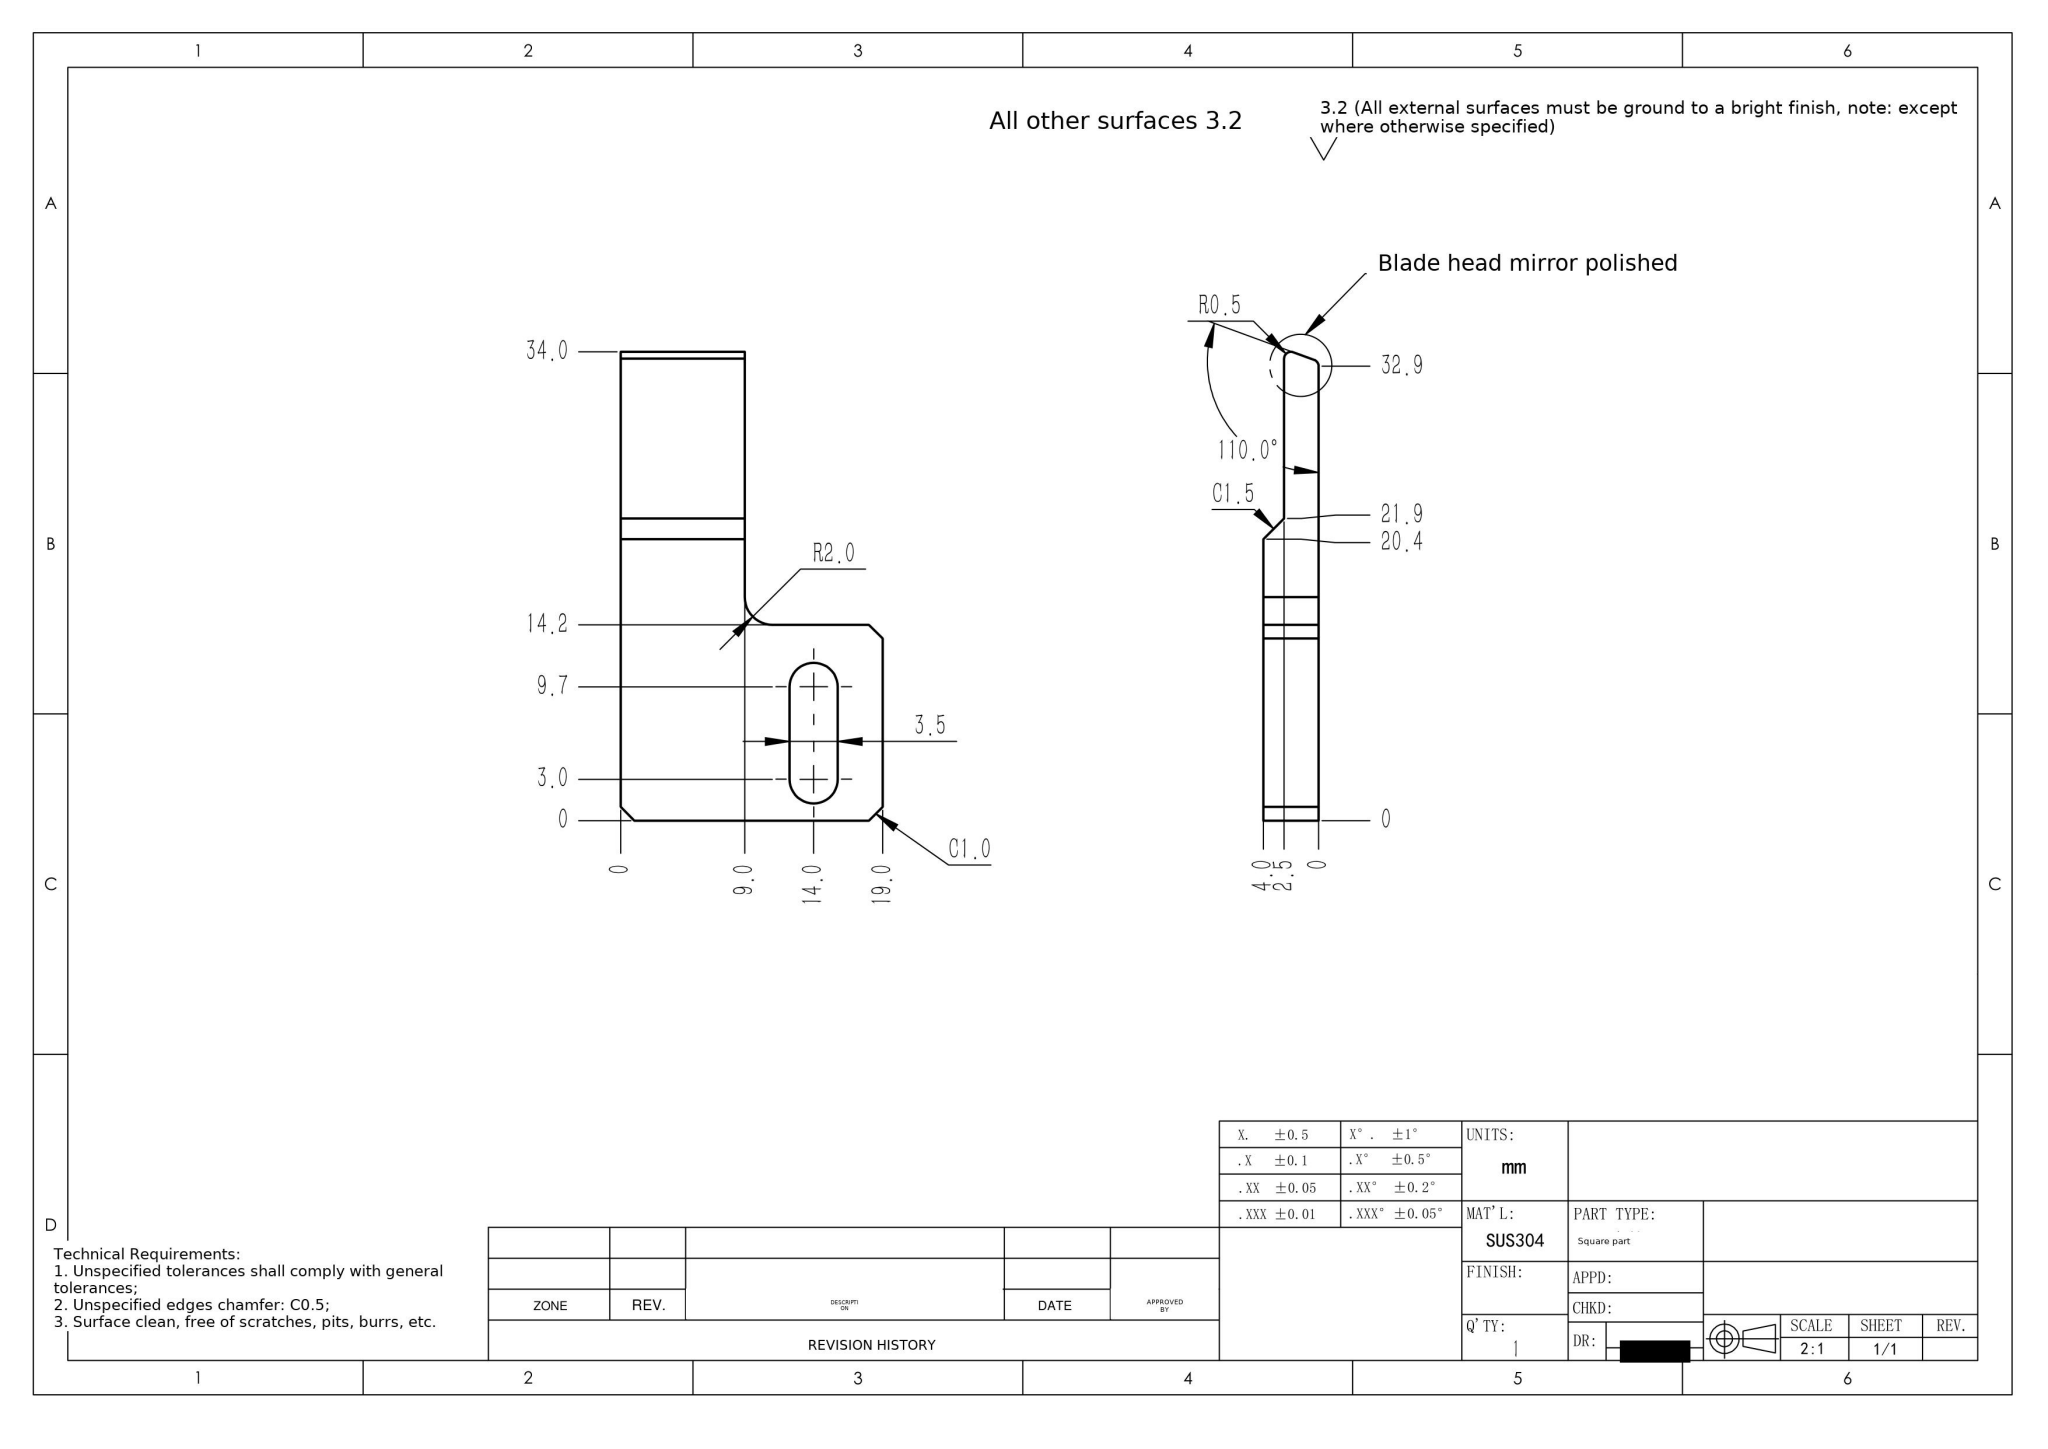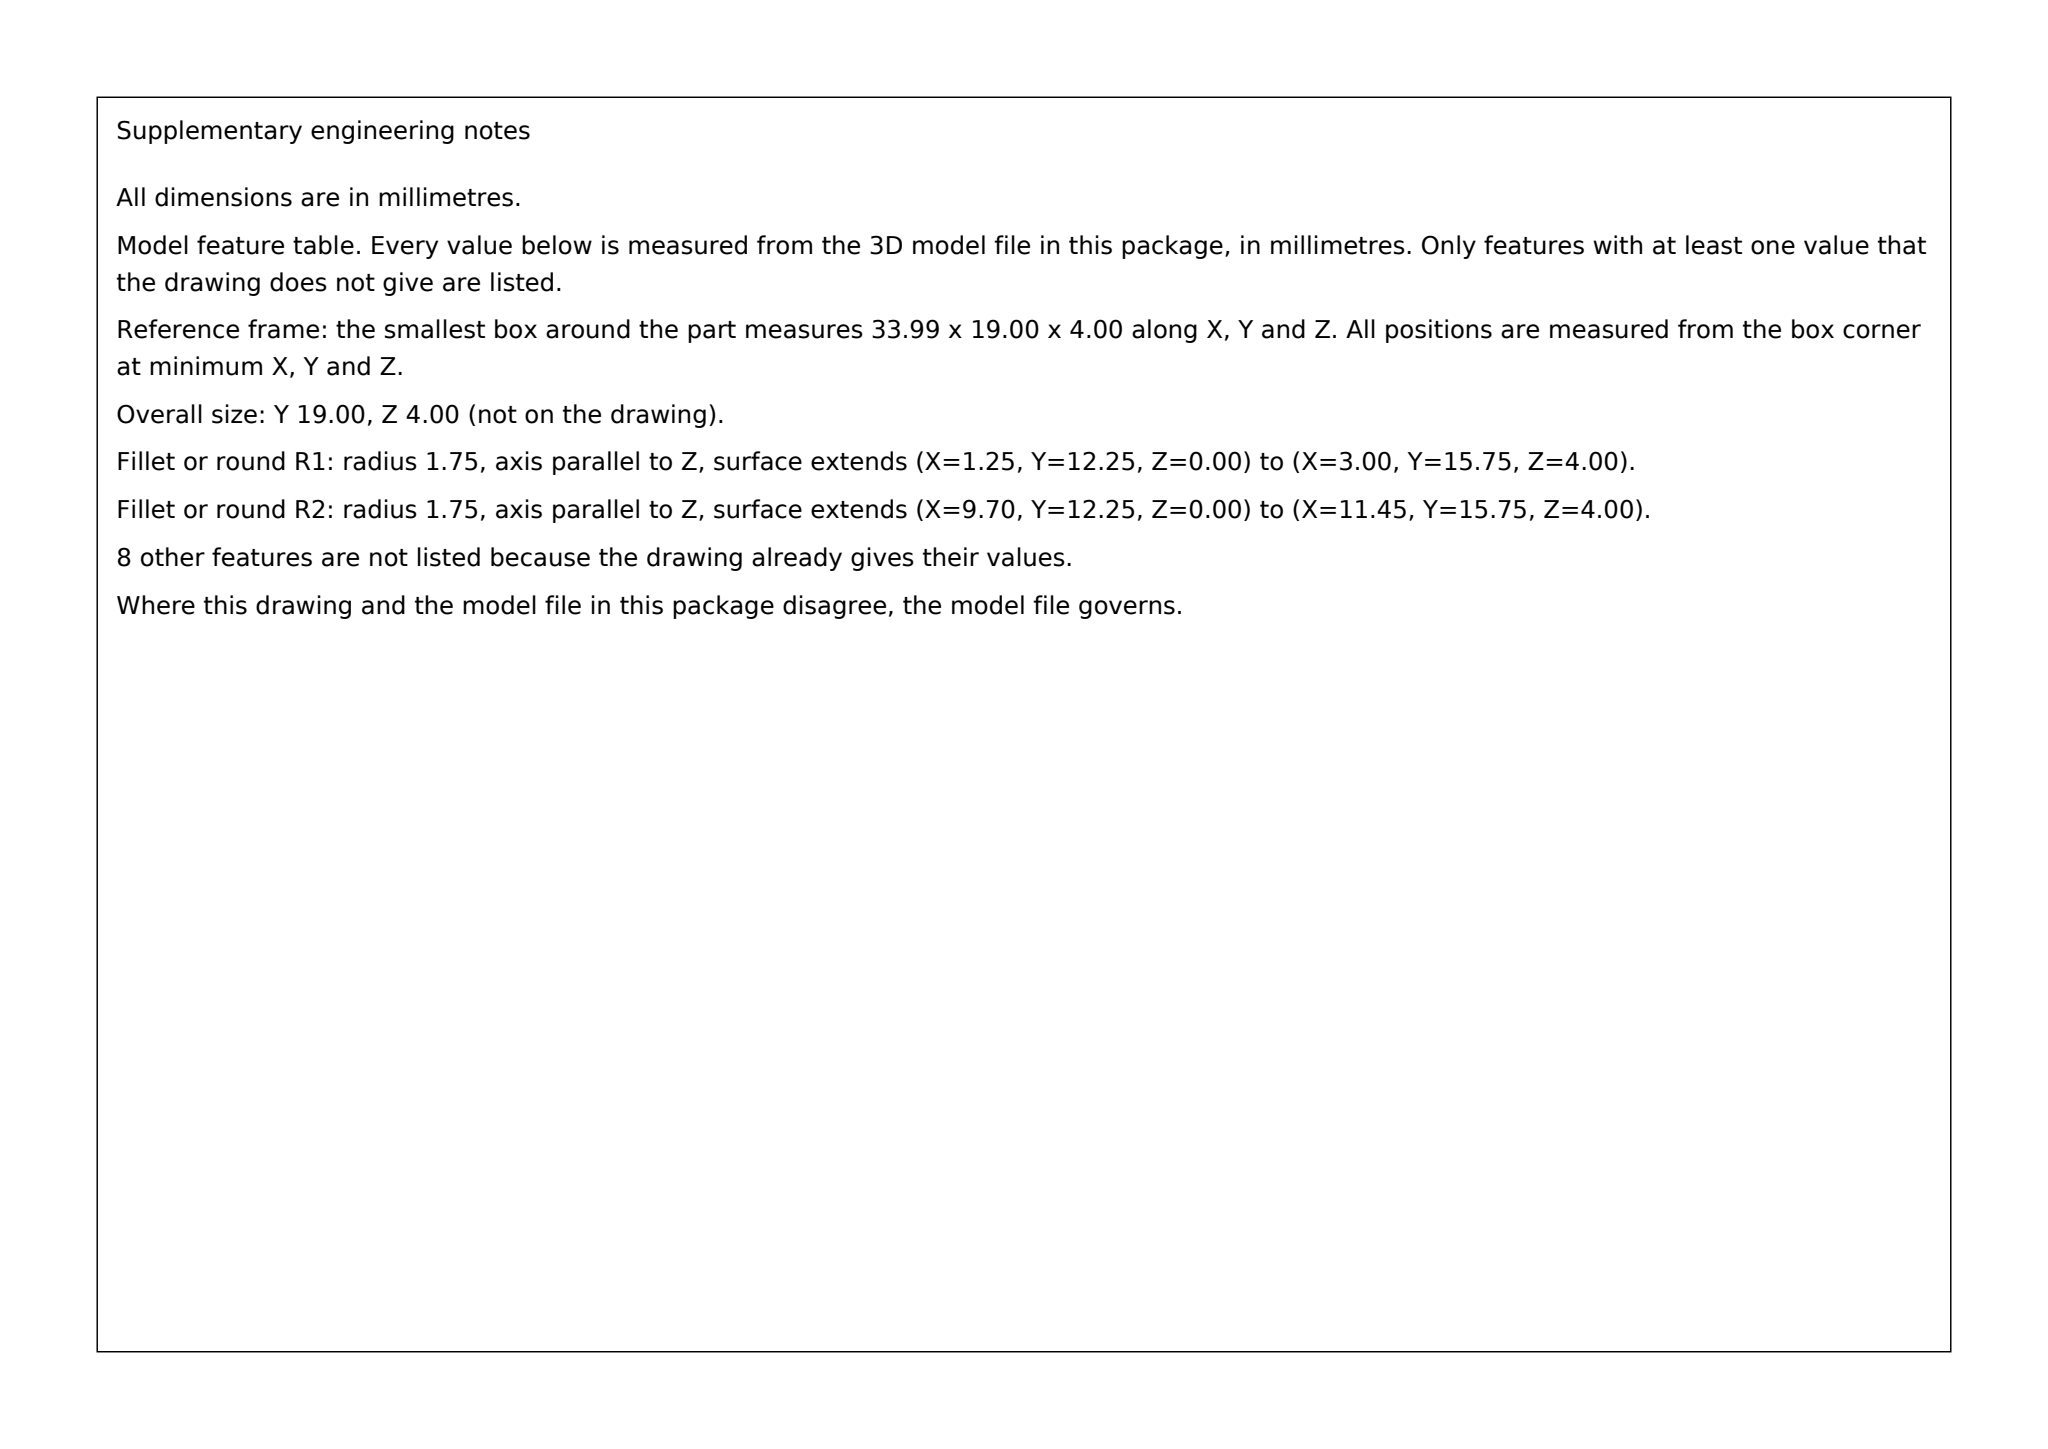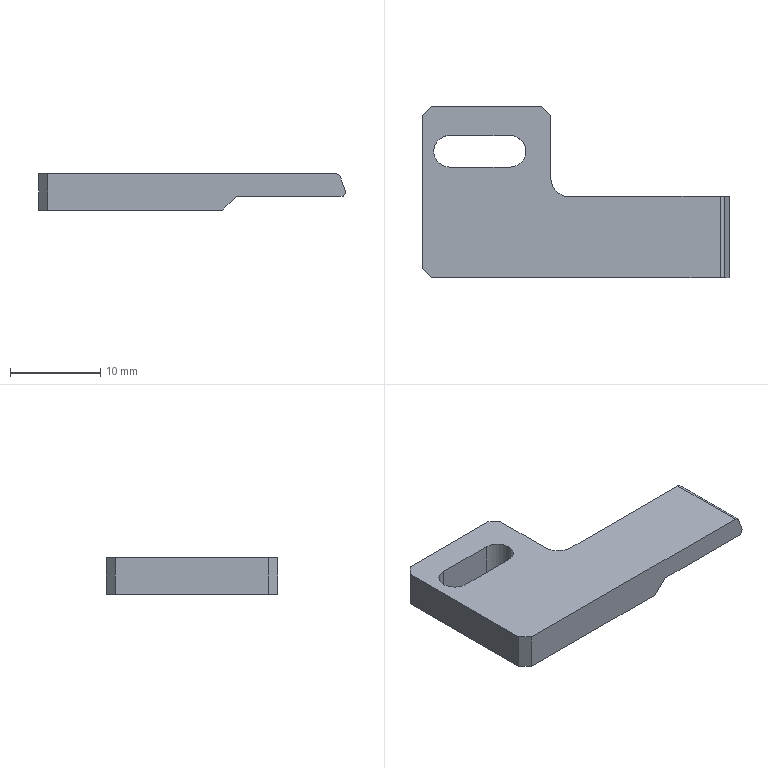Part | SolidWorks | mm | material SUS304 | 1 solid | 21 faces | box 33.99 x 19 x 4 mm | volume 1477 mm3 | plane 15 | cylinder 6 | commonest cylinder face diameters 3.5 x3 1 x2 4 x1
STEP:
#1=CARTESIAN_POINT('',(11.45,-5.,0.));
#2=VERTEX_POINT('',#1);
#3=CARTESIAN_POINT('',(9.7,-3.25,0.));
#4=VERTEX_POINT('',#3);
#5=CARTESIAN_POINT('',(9.7,-5.,0.));
#6=DIRECTION('',(0.,0.,1.));
#7=DIRECTION('',(1.,0.,0.));
#8=AXIS2_PLACEMENT_3D('',#5,#6,#7);
#9=CIRCLE('',#8,1.75);
#10=EDGE_CURVE('',#2,#4,#9,.T.);
#11=ORIENTED_EDGE('',*,*,#10,.F.);
#12=CARTESIAN_POINT('',(11.45,-5.,4.));
#13=VERTEX_POINT('',#12);
#14=CARTESIAN_POINT('',(11.45,-5.,0.));
#15=DIRECTION('',(0.,0.,1.));
#16=VECTOR('',#15,1000.);
#17=LINE('',#14,#16);
#18=EDGE_CURVE('',#2,#13,#17,.T.);
#19=ORIENTED_EDGE('',*,*,#18,.T.);
#20=CARTESIAN_POINT('',(9.7,-3.25,4.));
#21=VERTEX_POINT('',#20);
#22=CARTESIAN_POINT('',(9.7,-5.,4.));
#23=DIRECTION('',(0.,0.,1.));
#24=DIRECTION('',(1.,0.,0.));
#25=AXIS2_PLACEMENT_3D('',#22,#23,#24);
#26=CIRCLE('',#25,1.75);
#27=EDGE_CURVE('',#13,#21,#26,.T.);
#28=ORIENTED_EDGE('',*,*,#27,.T.);
#29=CARTESIAN_POINT('',(9.7,-3.25,0.));
#30=DIRECTION('',(0.,0.,1.));
#31=VECTOR('',#30,1000.);
#32=LINE('',#29,#31);
#33=EDGE_CURVE('',#4,#21,#32,.T.);
#34=ORIENTED_EDGE('',*,*,#33,.F.);
#35=EDGE_LOOP('',(#11,#19,#28,#34));
#36=FACE_OUTER_BOUND('',#35,.T.);
#37=CARTESIAN_POINT('',(9.7,-5.,0.));
#38=DIRECTION('',(0.,0.,1.));
#39=DIRECTION('',(1.,0.,0.));
#40=AXIS2_PLACEMENT_3D('',#37,#38,#39);
#41=CYLINDRICAL_SURFACE('',#40,1.75);
#42=ADVANCED_FACE('',(#36),#41,.F.);
#43=CARTESIAN_POINT('',(0.,-1.,4.));
#44=VERTEX_POINT('',#43);
#45=CARTESIAN_POINT('',(0.,-18.,4.));
#46=VERTEX_POINT('',#45);
#47=CARTESIAN_POINT('',(0.,0.,4.));
#48=DIRECTION('',(0.,-1.,0.));
#49=VECTOR('',#48,1000.);
#50=LINE('',#47,#49);
#51=EDGE_CURVE('',#44,#46,#50,.T.);
#52=ORIENTED_EDGE('',*,*,#51,.F.);
#53=CARTESIAN_POINT('',(0.,-1.,0.));
#54=VERTEX_POINT('',#53);
#55=CARTESIAN_POINT('',(0.,-1.,4.));
#56=DIRECTION('',(0.,0.,-1.));
#57=VECTOR('',#56,1000.);
#58=LINE('',#55,#57);
#59=EDGE_CURVE('',#44,#54,#58,.T.);
#60=ORIENTED_EDGE('',*,*,#59,.T.);
#61=CARTESIAN_POINT('',(0.,-18.,0.));
#62=VERTEX_POINT('',#61);
#63=CARTESIAN_POINT('',(0.,0.,0.));
#64=DIRECTION('',(0.,-1.,0.));
#65=VECTOR('',#64,1000.);
#66=LINE('',#63,#65);
#67=EDGE_CURVE('',#54,#62,#66,.T.);
#68=ORIENTED_EDGE('',*,*,#67,.T.);
#69=CARTESIAN_POINT('',(0.,-18.,4.));
#70=DIRECTION('',(0.,0.,1.));
#71=VECTOR('',#70,1000.);
#72=LINE('',#69,#71);
#73=EDGE_CURVE('',#62,#46,#72,.T.);
#74=ORIENTED_EDGE('',*,*,#73,.T.);
#75=EDGE_LOOP('',(#52,#60,#68,#74));
#76=FACE_OUTER_BOUND('',#75,.T.);
#77=CARTESIAN_POINT('',(0.,0.,4.));
#78=DIRECTION('',(1.,0.,0.));
#79=DIRECTION('',(0.,0.,-1.));
#80=AXIS2_PLACEMENT_3D('',#77,#78,#79);
#81=PLANE('',#80);
#82=ADVANCED_FACE('',(#76),#81,.F.);
#83=CARTESIAN_POINT('',(1.,-19.,4.));
#84=VERTEX_POINT('',#83);
#85=CARTESIAN_POINT('',(32.94,-19.,4.));
#86=VERTEX_POINT('',#85);
#87=CARTESIAN_POINT('',(0.,-19.,4.));
#88=DIRECTION('',(1.,0.,0.));
#89=VECTOR('',#88,1000.);
#90=LINE('',#87,#89);
#91=EDGE_CURVE('',#84,#86,#90,.T.);
#92=ORIENTED_EDGE('',*,*,#91,.F.);
#93=CARTESIAN_POINT('',(1.,-19.,0.));
#94=VERTEX_POINT('',#93);
#95=CARTESIAN_POINT('',(1.,-19.,4.));
#96=DIRECTION('',(0.,0.,-1.));
#97=VECTOR('',#96,1000.);
#98=LINE('',#95,#97);
#99=EDGE_CURVE('',#84,#94,#98,.T.);
#100=ORIENTED_EDGE('',*,*,#99,.T.);
#101=CARTESIAN_POINT('',(20.4,-19.,0.));
#102=VERTEX_POINT('',#101);
#103=CARTESIAN_POINT('',(0.,-19.,0.));
#104=DIRECTION('',(1.,0.,0.));
#105=VECTOR('',#104,1000.);
#106=LINE('',#103,#105);
#107=EDGE_CURVE('',#94,#102,#106,.T.);
#108=ORIENTED_EDGE('',*,*,#107,.T.);
#109=CARTESIAN_POINT('',(21.9,-19.,1.5));
#110=VERTEX_POINT('',#109);
#111=CARTESIAN_POINT('',(12.2,-19.,-8.2));
#112=DIRECTION('',(0.7071,0.,0.7071));
#113=VECTOR('',#112,1000.);
#114=LINE('',#111,#113);
#115=EDGE_CURVE('',#102,#110,#114,.T.);
#116=ORIENTED_EDGE('',*,*,#115,.T.);
#117=CARTESIAN_POINT('',(33.486,-19.,1.5));
#118=VERTEX_POINT('',#117);
#119=CARTESIAN_POINT('',(34.2,-19.,1.5));
#120=DIRECTION('',(-1.,0.,-0.));
#121=VECTOR('',#120,1000.);
#122=LINE('',#119,#121);
#123=EDGE_CURVE('',#118,#110,#122,.T.);
#124=ORIENTED_EDGE('',*,*,#123,.F.);
#125=CARTESIAN_POINT('',(33.956,-19.,2.171));
#126=VERTEX_POINT('',#125);
#127=CARTESIAN_POINT('',(33.486,-19.,2.));
#128=DIRECTION('',(0.,-1.,0.));
#129=DIRECTION('',(-0.,0.,1.));
#130=AXIS2_PLACEMENT_3D('',#127,#128,#129);
#131=CIRCLE('',#130,0.5);
#132=EDGE_CURVE('',#118,#126,#131,.T.);
#133=ORIENTED_EDGE('',*,*,#132,.T.);
#134=CARTESIAN_POINT('',(33.41,-19.,3.671));
#135=VERTEX_POINT('',#134);
#136=CARTESIAN_POINT('',(34.2,-19.,1.5));
#137=DIRECTION('',(0.342,0.,-0.9397));
#138=VECTOR('',#137,1000.);
#139=LINE('',#136,#138);
#140=EDGE_CURVE('',#135,#126,#139,.T.);
#141=ORIENTED_EDGE('',*,*,#140,.F.);
#142=CARTESIAN_POINT('',(32.94,-19.,3.5));
#143=DIRECTION('',(0.,-1.,0.));
#144=DIRECTION('',(0.,0.,1.));
#145=AXIS2_PLACEMENT_3D('',#142,#143,#144);
#146=CIRCLE('',#145,0.5);
#147=EDGE_CURVE('',#135,#86,#146,.T.);
#148=ORIENTED_EDGE('',*,*,#147,.T.);
#149=EDGE_LOOP('',(#92,#100,#108,#116,#124,#133,#141,#148));
#150=FACE_OUTER_BOUND('',#149,.T.);
#151=CARTESIAN_POINT('',(0.,-19.,4.));
#152=DIRECTION('',(0.,1.,0.));
#153=DIRECTION('',(0.,0.,1.));
#154=AXIS2_PLACEMENT_3D('',#151,#152,#153);
#155=PLANE('',#154);
#156=ADVANCED_FACE('',(#150),#155,.F.);
#157=CARTESIAN_POINT('',(13.2,0.,4.));
#158=VERTEX_POINT('',#157);
#159=CARTESIAN_POINT('',(1.,0.,4.));
#160=VERTEX_POINT('',#159);
#161=CARTESIAN_POINT('',(0.,0.,4.));
#162=DIRECTION('',(-1.,0.,0.));
#163=VECTOR('',#162,1000.);
#164=LINE('',#161,#163);
#165=EDGE_CURVE('',#158,#160,#164,.T.);
#166=ORIENTED_EDGE('',*,*,#165,.F.);
#167=CARTESIAN_POINT('',(13.2,0.,0.));
#168=VERTEX_POINT('',#167);
#169=CARTESIAN_POINT('',(13.2,0.,4.));
#170=DIRECTION('',(0.,0.,-1.));
#171=VECTOR('',#170,1000.);
#172=LINE('',#169,#171);
#173=EDGE_CURVE('',#158,#168,#172,.T.);
#174=ORIENTED_EDGE('',*,*,#173,.T.);
#175=CARTESIAN_POINT('',(1.,0.,0.));
#176=VERTEX_POINT('',#175);
#177=CARTESIAN_POINT('',(0.,0.,0.));
#178=DIRECTION('',(-1.,0.,0.));
#179=VECTOR('',#178,1000.);
#180=LINE('',#177,#179);
#181=EDGE_CURVE('',#168,#176,#180,.T.);
#182=ORIENTED_EDGE('',*,*,#181,.T.);
#183=CARTESIAN_POINT('',(1.,0.,4.));
#184=DIRECTION('',(0.,0.,1.));
#185=VECTOR('',#184,1000.);
#186=LINE('',#183,#185);
#187=EDGE_CURVE('',#176,#160,#186,.T.);
#188=ORIENTED_EDGE('',*,*,#187,.T.);
#189=EDGE_LOOP('',(#166,#174,#182,#188));
#190=FACE_OUTER_BOUND('',#189,.T.);
#191=CARTESIAN_POINT('',(0.,0.,4.));
#192=DIRECTION('',(0.,-1.,0.));
#193=DIRECTION('',(0.,0.,-1.));
#194=AXIS2_PLACEMENT_3D('',#191,#192,#193);
#195=PLANE('',#194);
#196=ADVANCED_FACE('',(#190),#195,.F.);
#197=CARTESIAN_POINT('',(14.2,-1.,4.));
#198=VERTEX_POINT('',#197);
#199=CARTESIAN_POINT('',(14.2,-8.,4.));
#200=VERTEX_POINT('',#199);
#201=CARTESIAN_POINT('',(14.2,-0.,4.));
#202=DIRECTION('',(0.,-1.,0.));
#203=VECTOR('',#202,1000.);
#204=LINE('',#201,#203);
#205=EDGE_CURVE('',#198,#200,#204,.T.);
#206=ORIENTED_EDGE('',*,*,#205,.F.);
#207=CARTESIAN_POINT('',(6.6,6.6,4.));
#208=DIRECTION('',(-0.7071,0.7071,0.));
#209=VECTOR('',#208,1000.);
#210=LINE('',#207,#209);
#211=EDGE_CURVE('',#198,#158,#210,.T.);
#212=ORIENTED_EDGE('',*,*,#211,.T.);
#213=ORIENTED_EDGE('',*,*,#165,.T.);
#214=CARTESIAN_POINT('',(0.5,-0.5,4.));
#215=DIRECTION('',(-0.7071,-0.7071,0.));
#216=VECTOR('',#215,1000.);
#217=LINE('',#214,#216);
#218=EDGE_CURVE('',#160,#44,#217,.T.);
#219=ORIENTED_EDGE('',*,*,#218,.T.);
#220=ORIENTED_EDGE('',*,*,#51,.T.);
#221=CARTESIAN_POINT('',(-9.,-9.,4.));
#222=DIRECTION('',(0.7071,-0.7071,0.));
#223=VECTOR('',#222,1000.);
#224=LINE('',#221,#223);
#225=EDGE_CURVE('',#46,#84,#224,.T.);
#226=ORIENTED_EDGE('',*,*,#225,.T.);
#227=ORIENTED_EDGE('',*,*,#91,.T.);
#228=CARTESIAN_POINT('',(32.94,-10.,4.));
#229=VERTEX_POINT('',#228);
#230=CARTESIAN_POINT('',(32.94,-10.,4.));
#231=DIRECTION('',(0.,1.,0.));
#232=VECTOR('',#231,1000.);
#233=LINE('',#230,#232);
#234=EDGE_CURVE('',#86,#229,#233,.T.);
#235=ORIENTED_EDGE('',*,*,#234,.T.);
#236=CARTESIAN_POINT('',(16.2,-10.,4.));
#237=VERTEX_POINT('',#236);
#238=CARTESIAN_POINT('',(34.2,-10.,4.));
#239=DIRECTION('',(1.,0.,0.));
#240=VECTOR('',#239,1000.);
#241=LINE('',#238,#240);
#242=EDGE_CURVE('',#237,#229,#241,.T.);
#243=ORIENTED_EDGE('',*,*,#242,.F.);
#244=CARTESIAN_POINT('',(16.2,-8.,4.));
#245=DIRECTION('',(0.,0.,-1.));
#246=DIRECTION('',(1.,0.,0.));
#247=AXIS2_PLACEMENT_3D('',#244,#245,#246);
#248=CIRCLE('',#247,2.);
#249=EDGE_CURVE('',#237,#200,#248,.T.);
#250=ORIENTED_EDGE('',*,*,#249,.T.);
#251=EDGE_LOOP('',(#206,#212,#213,#219,#220,#226,#227,#235,#243,#250));
#252=FACE_OUTER_BOUND('',#251,.T.);
#253=CARTESIAN_POINT('',(3.,-3.25,4.));
#254=VERTEX_POINT('',#253);
#255=CARTESIAN_POINT('',(3.,-6.75,4.));
#256=VERTEX_POINT('',#255);
#257=CARTESIAN_POINT('',(3.,-5.,4.));
#258=DIRECTION('',(0.,0.,1.));
#259=DIRECTION('',(1.,0.,0.));
#260=AXIS2_PLACEMENT_3D('',#257,#258,#259);
#261=CIRCLE('',#260,1.75);
#262=EDGE_CURVE('',#254,#256,#261,.T.);
#263=ORIENTED_EDGE('',*,*,#262,.F.);
#264=CARTESIAN_POINT('',(3.,-3.25,4.));
#265=DIRECTION('',(-1.,0.,0.));
#266=VECTOR('',#265,1000.);
#267=LINE('',#264,#266);
#268=EDGE_CURVE('',#21,#254,#267,.T.);
#269=ORIENTED_EDGE('',*,*,#268,.F.);
#270=ORIENTED_EDGE('',*,*,#27,.F.);
#271=CARTESIAN_POINT('',(9.7,-6.75,4.));
#272=VERTEX_POINT('',#271);
#273=CARTESIAN_POINT('',(9.7,-5.,4.));
#274=DIRECTION('',(0.,0.,1.));
#275=DIRECTION('',(1.,0.,0.));
#276=AXIS2_PLACEMENT_3D('',#273,#274,#275);
#277=CIRCLE('',#276,1.75);
#278=EDGE_CURVE('',#272,#13,#277,.T.);
#279=ORIENTED_EDGE('',*,*,#278,.F.);
#280=CARTESIAN_POINT('',(3.,-6.75,4.));
#281=DIRECTION('',(1.,0.,0.));
#282=VECTOR('',#281,1000.);
#283=LINE('',#280,#282);
#284=EDGE_CURVE('',#256,#272,#283,.T.);
#285=ORIENTED_EDGE('',*,*,#284,.F.);
#286=EDGE_LOOP('',(#263,#269,#270,#279,#285));
#287=FACE_BOUND('',#286,.T.);
#288=CARTESIAN_POINT('',(0.,0.,4.));
#289=DIRECTION('',(0.,0.,1.));
#290=DIRECTION('',(1.,0.,0.));
#291=AXIS2_PLACEMENT_3D('',#288,#289,#290);
#292=PLANE('',#291);
#293=ADVANCED_FACE('',(#252,#287),#292,.T.);
#294=CARTESIAN_POINT('',(3.,-3.25,0.));
#295=VERTEX_POINT('',#294);
#296=CARTESIAN_POINT('',(3.,-3.25,0.));
#297=DIRECTION('',(-1.,0.,0.));
#298=VECTOR('',#297,1000.);
#299=LINE('',#296,#298);
#300=EDGE_CURVE('',#4,#295,#299,.T.);
#301=ORIENTED_EDGE('',*,*,#300,.T.);
#302=CARTESIAN_POINT('',(3.,-6.75,0.));
#303=VERTEX_POINT('',#302);
#304=CARTESIAN_POINT('',(3.,-5.,0.));
#305=DIRECTION('',(0.,0.,1.));
#306=DIRECTION('',(1.,0.,0.));
#307=AXIS2_PLACEMENT_3D('',#304,#305,#306);
#308=CIRCLE('',#307,1.75);
#309=EDGE_CURVE('',#295,#303,#308,.T.);
#310=ORIENTED_EDGE('',*,*,#309,.T.);
#311=CARTESIAN_POINT('',(9.7,-6.75,0.));
#312=VERTEX_POINT('',#311);
#313=CARTESIAN_POINT('',(3.,-6.75,0.));
#314=DIRECTION('',(1.,0.,0.));
#315=VECTOR('',#314,1000.);
#316=LINE('',#313,#315);
#317=EDGE_CURVE('',#303,#312,#316,.T.);
#318=ORIENTED_EDGE('',*,*,#317,.T.);
#319=CARTESIAN_POINT('',(9.7,-5.,0.));
#320=DIRECTION('',(0.,0.,1.));
#321=DIRECTION('',(1.,0.,0.));
#322=AXIS2_PLACEMENT_3D('',#319,#320,#321);
#323=CIRCLE('',#322,1.75);
#324=EDGE_CURVE('',#312,#2,#323,.T.);
#325=ORIENTED_EDGE('',*,*,#324,.T.);
#326=ORIENTED_EDGE('',*,*,#10,.T.);
#327=EDGE_LOOP('',(#301,#310,#318,#325,#326));
#328=FACE_BOUND('',#327,.T.);
#329=ORIENTED_EDGE('',*,*,#181,.F.);
#330=CARTESIAN_POINT('',(14.2,-1.,0.));
#331=VERTEX_POINT('',#330);
#332=CARTESIAN_POINT('',(14.2,-1.,0.));
#333=DIRECTION('',(0.7071,-0.7071,0.));
#334=VECTOR('',#333,1000.);
#335=LINE('',#332,#334);
#336=EDGE_CURVE('',#168,#331,#335,.T.);
#337=ORIENTED_EDGE('',*,*,#336,.T.);
#338=CARTESIAN_POINT('',(14.2,-8.,0.));
#339=VERTEX_POINT('',#338);
#340=CARTESIAN_POINT('',(14.2,-0.,0.));
#341=DIRECTION('',(0.,-1.,0.));
#342=VECTOR('',#341,1000.);
#343=LINE('',#340,#342);
#344=EDGE_CURVE('',#331,#339,#343,.T.);
#345=ORIENTED_EDGE('',*,*,#344,.T.);
#346=CARTESIAN_POINT('',(16.2,-10.,0.));
#347=VERTEX_POINT('',#346);
#348=CARTESIAN_POINT('',(16.2,-8.,0.));
#349=DIRECTION('',(0.,0.,1.));
#350=DIRECTION('',(1.,0.,0.));
#351=AXIS2_PLACEMENT_3D('',#348,#349,#350);
#352=CIRCLE('',#351,2.);
#353=EDGE_CURVE('',#339,#347,#352,.T.);
#354=ORIENTED_EDGE('',*,*,#353,.T.);
#355=CARTESIAN_POINT('',(20.4,-10.,0.));
#356=VERTEX_POINT('',#355);
#357=CARTESIAN_POINT('',(34.2,-10.,0.));
#358=DIRECTION('',(1.,0.,0.));
#359=VECTOR('',#358,1000.);
#360=LINE('',#357,#359);
#361=EDGE_CURVE('',#347,#356,#360,.T.);
#362=ORIENTED_EDGE('',*,*,#361,.T.);
#363=CARTESIAN_POINT('',(20.4,0.,0.));
#364=DIRECTION('',(0.,-1.,0.));
#365=VECTOR('',#364,1000.);
#366=LINE('',#363,#365);
#367=EDGE_CURVE('',#356,#102,#366,.T.);
#368=ORIENTED_EDGE('',*,*,#367,.T.);
#369=ORIENTED_EDGE('',*,*,#107,.F.);
#370=CARTESIAN_POINT('',(1.,-19.,0.));
#371=DIRECTION('',(-0.7071,0.7071,0.));
#372=VECTOR('',#371,1000.);
#373=LINE('',#370,#372);
#374=EDGE_CURVE('',#94,#62,#373,.T.);
#375=ORIENTED_EDGE('',*,*,#374,.T.);
#376=ORIENTED_EDGE('',*,*,#67,.F.);
#377=CARTESIAN_POINT('',(0.,-1.,0.));
#378=DIRECTION('',(0.7071,0.7071,0.));
#379=VECTOR('',#378,1000.);
#380=LINE('',#377,#379);
#381=EDGE_CURVE('',#54,#176,#380,.T.);
#382=ORIENTED_EDGE('',*,*,#381,.T.);
#383=EDGE_LOOP('',(#329,#337,#345,#354,#362,#368,#369,#375,#376,#382));
#384=FACE_OUTER_BOUND('',#383,.T.);
#385=CARTESIAN_POINT('',(0.,0.,0.));
#386=DIRECTION('',(0.,0.,1.));
#387=DIRECTION('',(1.,0.,0.));
#388=AXIS2_PLACEMENT_3D('',#385,#386,#387);
#389=PLANE('',#388);
#390=ADVANCED_FACE('',(#328,#384),#389,.F.);
#391=ORIENTED_EDGE('',*,*,#262,.T.);
#392=CARTESIAN_POINT('',(3.,-6.75,0.));
#393=DIRECTION('',(0.,0.,1.));
#394=VECTOR('',#393,1000.);
#395=LINE('',#392,#394);
#396=EDGE_CURVE('',#303,#256,#395,.T.);
#397=ORIENTED_EDGE('',*,*,#396,.F.);
#398=ORIENTED_EDGE('',*,*,#309,.F.);
#399=CARTESIAN_POINT('',(3.,-3.25,0.));
#400=DIRECTION('',(0.,0.,1.));
#401=VECTOR('',#400,1000.);
#402=LINE('',#399,#401);
#403=EDGE_CURVE('',#295,#254,#402,.T.);
#404=ORIENTED_EDGE('',*,*,#403,.T.);
#405=EDGE_LOOP('',(#391,#397,#398,#404));
#406=FACE_OUTER_BOUND('',#405,.T.);
#407=CARTESIAN_POINT('',(3.,-5.,0.));
#408=DIRECTION('',(0.,0.,1.));
#409=DIRECTION('',(1.,0.,0.));
#410=AXIS2_PLACEMENT_3D('',#407,#408,#409);
#411=CYLINDRICAL_SURFACE('',#410,1.75);
#412=ADVANCED_FACE('',(#406),#411,.F.);
#413=ORIENTED_EDGE('',*,*,#268,.T.);
#414=ORIENTED_EDGE('',*,*,#403,.F.);
#415=ORIENTED_EDGE('',*,*,#300,.F.);
#416=ORIENTED_EDGE('',*,*,#33,.T.);
#417=EDGE_LOOP('',(#413,#414,#415,#416));
#418=FACE_OUTER_BOUND('',#417,.T.);
#419=CARTESIAN_POINT('',(3.,-3.25,0.));
#420=DIRECTION('',(0.,1.,0.));
#421=DIRECTION('',(0.,0.,1.));
#422=AXIS2_PLACEMENT_3D('',#419,#420,#421);
#423=PLANE('',#422);
#424=ADVANCED_FACE('',(#418),#423,.F.);
#425=ORIENTED_EDGE('',*,*,#18,.F.);
#426=ORIENTED_EDGE('',*,*,#324,.F.);
#427=CARTESIAN_POINT('',(9.7,-6.75,0.));
#428=DIRECTION('',(0.,0.,1.));
#429=VECTOR('',#428,1000.);
#430=LINE('',#427,#429);
#431=EDGE_CURVE('',#312,#272,#430,.T.);
#432=ORIENTED_EDGE('',*,*,#431,.T.);
#433=ORIENTED_EDGE('',*,*,#278,.T.);
#434=EDGE_LOOP('',(#425,#426,#432,#433));
#435=FACE_OUTER_BOUND('',#434,.T.);
#436=CARTESIAN_POINT('',(9.7,-5.,0.));
#437=DIRECTION('',(0.,0.,1.));
#438=DIRECTION('',(1.,0.,0.));
#439=AXIS2_PLACEMENT_3D('',#436,#437,#438);
#440=CYLINDRICAL_SURFACE('',#439,1.75);
#441=ADVANCED_FACE('',(#435),#440,.F.);
#442=ORIENTED_EDGE('',*,*,#284,.T.);
#443=ORIENTED_EDGE('',*,*,#431,.F.);
#444=ORIENTED_EDGE('',*,*,#317,.F.);
#445=ORIENTED_EDGE('',*,*,#396,.T.);
#446=EDGE_LOOP('',(#442,#443,#444,#445));
#447=FACE_OUTER_BOUND('',#446,.T.);
#448=CARTESIAN_POINT('',(3.,-6.75,0.));
#449=DIRECTION('',(0.,-1.,0.));
#450=DIRECTION('',(0.,0.,-1.));
#451=AXIS2_PLACEMENT_3D('',#448,#449,#450);
#452=PLANE('',#451);
#453=ADVANCED_FACE('',(#447),#452,.F.);
#454=ORIENTED_EDGE('',*,*,#361,.F.);
#455=CARTESIAN_POINT('',(16.2,-10.,4.));
#456=DIRECTION('',(0.,0.,1.));
#457=VECTOR('',#456,1000.);
#458=LINE('',#455,#457);
#459=EDGE_CURVE('',#347,#237,#458,.T.);
#460=ORIENTED_EDGE('',*,*,#459,.T.);
#461=ORIENTED_EDGE('',*,*,#242,.T.);
#462=CARTESIAN_POINT('',(33.41,-10.,3.671));
#463=VERTEX_POINT('',#462);
#464=CARTESIAN_POINT('',(32.94,-10.,3.5));
#465=DIRECTION('',(-0.,1.,0.));
#466=DIRECTION('',(1.,0.,0.));
#467=AXIS2_PLACEMENT_3D('',#464,#465,#466);
#468=CIRCLE('',#467,0.5);
#469=EDGE_CURVE('',#229,#463,#468,.T.);
#470=ORIENTED_EDGE('',*,*,#469,.T.);
#471=CARTESIAN_POINT('',(33.956,-10.,2.171));
#472=VERTEX_POINT('',#471);
#473=CARTESIAN_POINT('',(34.682,-10.,0.1755));
#474=DIRECTION('',(0.342,0.,-0.9397));
#475=VECTOR('',#474,1000.);
#476=LINE('',#473,#475);
#477=EDGE_CURVE('',#463,#472,#476,.T.);
#478=ORIENTED_EDGE('',*,*,#477,.T.);
#479=CARTESIAN_POINT('',(33.486,-10.,1.5));
#480=VERTEX_POINT('',#479);
#481=CARTESIAN_POINT('',(33.486,-10.,2.));
#482=DIRECTION('',(-0.,1.,0.));
#483=DIRECTION('',(1.,0.,-0.));
#484=AXIS2_PLACEMENT_3D('',#481,#482,#483);
#485=CIRCLE('',#484,0.5);
#486=EDGE_CURVE('',#472,#480,#485,.T.);
#487=ORIENTED_EDGE('',*,*,#486,.T.);
#488=CARTESIAN_POINT('',(21.9,-10.,1.5));
#489=VERTEX_POINT('',#488);
#490=CARTESIAN_POINT('',(34.2,-10.,1.5));
#491=DIRECTION('',(-1.,-0.,-0.));
#492=VECTOR('',#491,1000.);
#493=LINE('',#490,#492);
#494=EDGE_CURVE('',#480,#489,#493,.T.);
#495=ORIENTED_EDGE('',*,*,#494,.T.);
#496=CARTESIAN_POINT('',(27.3,-10.,6.9));
#497=DIRECTION('',(-0.7071,-0.,-0.7071));
#498=VECTOR('',#497,1000.);
#499=LINE('',#496,#498);
#500=EDGE_CURVE('',#489,#356,#499,.T.);
#501=ORIENTED_EDGE('',*,*,#500,.T.);
#502=EDGE_LOOP('',(#454,#460,#461,#470,#478,#487,#495,#501));
#503=FACE_OUTER_BOUND('',#502,.T.);
#504=CARTESIAN_POINT('',(34.2,-10.,0.));
#505=DIRECTION('',(0.,-1.,0.));
#506=DIRECTION('',(1.,0.,0.));
#507=AXIS2_PLACEMENT_3D('',#504,#505,#506);
#508=PLANE('',#507);
#509=ADVANCED_FACE('',(#503),#508,.F.);
#510=ORIENTED_EDGE('',*,*,#205,.T.);
#511=CARTESIAN_POINT('',(14.2,-8.,0.));
#512=DIRECTION('',(0.,0.,-1.));
#513=VECTOR('',#512,1000.);
#514=LINE('',#511,#513);
#515=EDGE_CURVE('',#200,#339,#514,.T.);
#516=ORIENTED_EDGE('',*,*,#515,.T.);
#517=ORIENTED_EDGE('',*,*,#344,.F.);
#518=CARTESIAN_POINT('',(14.2,-1.,0.));
#519=DIRECTION('',(0.,0.,1.));
#520=VECTOR('',#519,1000.);
#521=LINE('',#518,#520);
#522=EDGE_CURVE('',#331,#198,#521,.T.);
#523=ORIENTED_EDGE('',*,*,#522,.T.);
#524=EDGE_LOOP('',(#510,#516,#517,#523));
#525=FACE_OUTER_BOUND('',#524,.T.);
#526=CARTESIAN_POINT('',(14.2,-0.,0.));
#527=DIRECTION('',(-1.,-0.,0.));
#528=DIRECTION('',(0.,-1.,0.));
#529=AXIS2_PLACEMENT_3D('',#526,#527,#528);
#530=PLANE('',#529);
#531=ADVANCED_FACE('',(#525),#530,.F.);
#532=ORIENTED_EDGE('',*,*,#123,.T.);
#533=CARTESIAN_POINT('',(21.9,-10.,1.5));
#534=DIRECTION('',(0.,1.,0.));
#535=VECTOR('',#534,1000.);
#536=LINE('',#533,#535);
#537=EDGE_CURVE('',#110,#489,#536,.T.);
#538=ORIENTED_EDGE('',*,*,#537,.T.);
#539=ORIENTED_EDGE('',*,*,#494,.F.);
#540=CARTESIAN_POINT('',(33.486,0.,1.5));
#541=DIRECTION('',(0.,-1.,0.));
#542=VECTOR('',#541,1000.);
#543=LINE('',#540,#542);
#544=EDGE_CURVE('',#480,#118,#543,.T.);
#545=ORIENTED_EDGE('',*,*,#544,.T.);
#546=EDGE_LOOP('',(#532,#538,#539,#545));
#547=FACE_OUTER_BOUND('',#546,.T.);
#548=CARTESIAN_POINT('',(34.2,0.,1.5));
#549=DIRECTION('',(-0.,0.,1.));
#550=DIRECTION('',(1.,0.,0.));
#551=AXIS2_PLACEMENT_3D('',#548,#549,#550);
#552=PLANE('',#551);
#553=ADVANCED_FACE('',(#547),#552,.F.);
#554=ORIENTED_EDGE('',*,*,#140,.T.);
#555=CARTESIAN_POINT('',(33.956,0.,2.171));
#556=DIRECTION('',(0.,1.,0.));
#557=VECTOR('',#556,1000.);
#558=LINE('',#555,#557);
#559=EDGE_CURVE('',#126,#472,#558,.T.);
#560=ORIENTED_EDGE('',*,*,#559,.T.);
#561=ORIENTED_EDGE('',*,*,#477,.F.);
#562=CARTESIAN_POINT('',(33.41,-19.,3.671));
#563=DIRECTION('',(0.,-1.,0.));
#564=VECTOR('',#563,1000.);
#565=LINE('',#562,#564);
#566=EDGE_CURVE('',#463,#135,#565,.T.);
#567=ORIENTED_EDGE('',*,*,#566,.T.);
#568=EDGE_LOOP('',(#554,#560,#561,#567));
#569=FACE_OUTER_BOUND('',#568,.T.);
#570=CARTESIAN_POINT('',(34.2,0.,1.5));
#571=DIRECTION('',(-0.9397,0.,-0.342));
#572=DIRECTION('',(-0.342,0.,0.9397));
#573=AXIS2_PLACEMENT_3D('',#570,#571,#572);
#574=PLANE('',#573);
#575=ADVANCED_FACE('',(#569),#574,.F.);
#576=ORIENTED_EDGE('',*,*,#486,.F.);
#577=ORIENTED_EDGE('',*,*,#559,.F.);
#578=ORIENTED_EDGE('',*,*,#132,.F.);
#579=ORIENTED_EDGE('',*,*,#544,.F.);
#580=EDGE_LOOP('',(#576,#577,#578,#579));
#581=FACE_OUTER_BOUND('',#580,.T.);
#582=CARTESIAN_POINT('',(33.486,0.,2.));
#583=DIRECTION('',(0.,-1.,0.));
#584=DIRECTION('',(0.,0.,-1.));
#585=AXIS2_PLACEMENT_3D('',#582,#583,#584);
#586=CYLINDRICAL_SURFACE('',#585,0.5);
#587=ADVANCED_FACE('',(#581),#586,.T.);
#588=ORIENTED_EDGE('',*,*,#469,.F.);
#589=ORIENTED_EDGE('',*,*,#234,.F.);
#590=ORIENTED_EDGE('',*,*,#147,.F.);
#591=ORIENTED_EDGE('',*,*,#566,.F.);
#592=EDGE_LOOP('',(#588,#589,#590,#591));
#593=FACE_OUTER_BOUND('',#592,.T.);
#594=CARTESIAN_POINT('',(32.94,0.,3.5));
#595=DIRECTION('',(0.,1.,0.));
#596=DIRECTION('',(0.,0.,1.));
#597=AXIS2_PLACEMENT_3D('',#594,#595,#596);
#598=CYLINDRICAL_SURFACE('',#597,0.5);
#599=ADVANCED_FACE('',(#593),#598,.T.);
#600=ORIENTED_EDGE('',*,*,#500,.F.);
#601=ORIENTED_EDGE('',*,*,#537,.F.);
#602=ORIENTED_EDGE('',*,*,#115,.F.);
#603=ORIENTED_EDGE('',*,*,#367,.F.);
#604=EDGE_LOOP('',(#600,#601,#602,#603));
#605=FACE_OUTER_BOUND('',#604,.T.);
#606=CARTESIAN_POINT('',(20.2,0.,-0.2));
#607=DIRECTION('',(0.7071,0.,-0.7071));
#608=DIRECTION('',(0.,1.,0.));
#609=AXIS2_PLACEMENT_3D('',#606,#607,#608);
#610=PLANE('',#609);
#611=ADVANCED_FACE('',(#605),#610,.T.);
#612=ORIENTED_EDGE('',*,*,#336,.F.);
#613=ORIENTED_EDGE('',*,*,#173,.F.);
#614=ORIENTED_EDGE('',*,*,#211,.F.);
#615=ORIENTED_EDGE('',*,*,#522,.F.);
#616=EDGE_LOOP('',(#612,#613,#614,#615));
#617=FACE_OUTER_BOUND('',#616,.T.);
#618=CARTESIAN_POINT('',(14.2,-1.,0.));
#619=DIRECTION('',(-0.7071,-0.7071,0.));
#620=DIRECTION('',(0.,0.,1.));
#621=AXIS2_PLACEMENT_3D('',#618,#619,#620);
#622=PLANE('',#621);
#623=ADVANCED_FACE('',(#617),#622,.F.);
#624=ORIENTED_EDGE('',*,*,#218,.F.);
#625=ORIENTED_EDGE('',*,*,#187,.F.);
#626=ORIENTED_EDGE('',*,*,#381,.F.);
#627=ORIENTED_EDGE('',*,*,#59,.F.);
#628=EDGE_LOOP('',(#624,#625,#626,#627));
#629=FACE_OUTER_BOUND('',#628,.T.);
#630=CARTESIAN_POINT('',(0.,-1.,4.));
#631=DIRECTION('',(0.7071,-0.7071,0.));
#632=DIRECTION('',(0.,0.,-1.));
#633=AXIS2_PLACEMENT_3D('',#630,#631,#632);
#634=PLANE('',#633);
#635=ADVANCED_FACE('',(#629),#634,.F.);
#636=ORIENTED_EDGE('',*,*,#225,.F.);
#637=ORIENTED_EDGE('',*,*,#73,.F.);
#638=ORIENTED_EDGE('',*,*,#374,.F.);
#639=ORIENTED_EDGE('',*,*,#99,.F.);
#640=EDGE_LOOP('',(#636,#637,#638,#639));
#641=FACE_OUTER_BOUND('',#640,.T.);
#642=CARTESIAN_POINT('',(1.,-19.,4.));
#643=DIRECTION('',(0.7071,0.7071,0.));
#644=DIRECTION('',(0.,0.,-1.));
#645=AXIS2_PLACEMENT_3D('',#642,#643,#644);
#646=PLANE('',#645);
#647=ADVANCED_FACE('',(#641),#646,.F.);
#648=ORIENTED_EDGE('',*,*,#353,.F.);
#649=ORIENTED_EDGE('',*,*,#515,.F.);
#650=ORIENTED_EDGE('',*,*,#249,.F.);
#651=ORIENTED_EDGE('',*,*,#459,.F.);
#652=EDGE_LOOP('',(#648,#649,#650,#651));
#653=FACE_OUTER_BOUND('',#652,.T.);
#654=CARTESIAN_POINT('',(16.2,-8.,0.));
#655=DIRECTION('',(0.,0.,-1.));
#656=DIRECTION('',(-1.,0.,0.));
#657=AXIS2_PLACEMENT_3D('',#654,#655,#656);
#658=CYLINDRICAL_SURFACE('',#657,2.);
#659=ADVANCED_FACE('',(#653),#658,.F.);
#660=CLOSED_SHELL('',(#42,#82,#156,#196,#293,#390,#412,#424,#441,#453,#509,#531,#553,#575,#587,#599,#611,#623,#635,#647,#659));
#661=MANIFOLD_SOLID_BREP('',#660);
#662=CARTESIAN_POINT('',(0.,0.,0.));
#663=DIRECTION('',(0.,0.,1.));
#664=DIRECTION('',(1.,0.,0.));
#665=AXIS2_PLACEMENT_3D('',#662,#663,#664);
#666=(LENGTH_UNIT()NAMED_UNIT(*)SI_UNIT(.MILLI.,.METRE.));
#667=UNCERTAINTY_MEASURE_WITH_UNIT(LENGTH_MEASURE(0.00001),#666,'','');
#668=(NAMED_UNIT(*)PLANE_ANGLE_UNIT()SI_UNIT($,.RADIAN.));
#669=(NAMED_UNIT(*)SI_UNIT($,.STERADIAN.)SOLID_ANGLE_UNIT());
#670=(GEOMETRIC_REPRESENTATION_CONTEXT(3)GLOBAL_UNCERTAINTY_ASSIGNED_CONTEXT((#667))GLOBAL_UNIT_ASSIGNED_CONTEXT((#666,#668,#669))REPRESENTATION_CONTEXT('',''));
#671=ADVANCED_BREP_SHAPE_REPRESENTATION('',(#661,#665),#670);